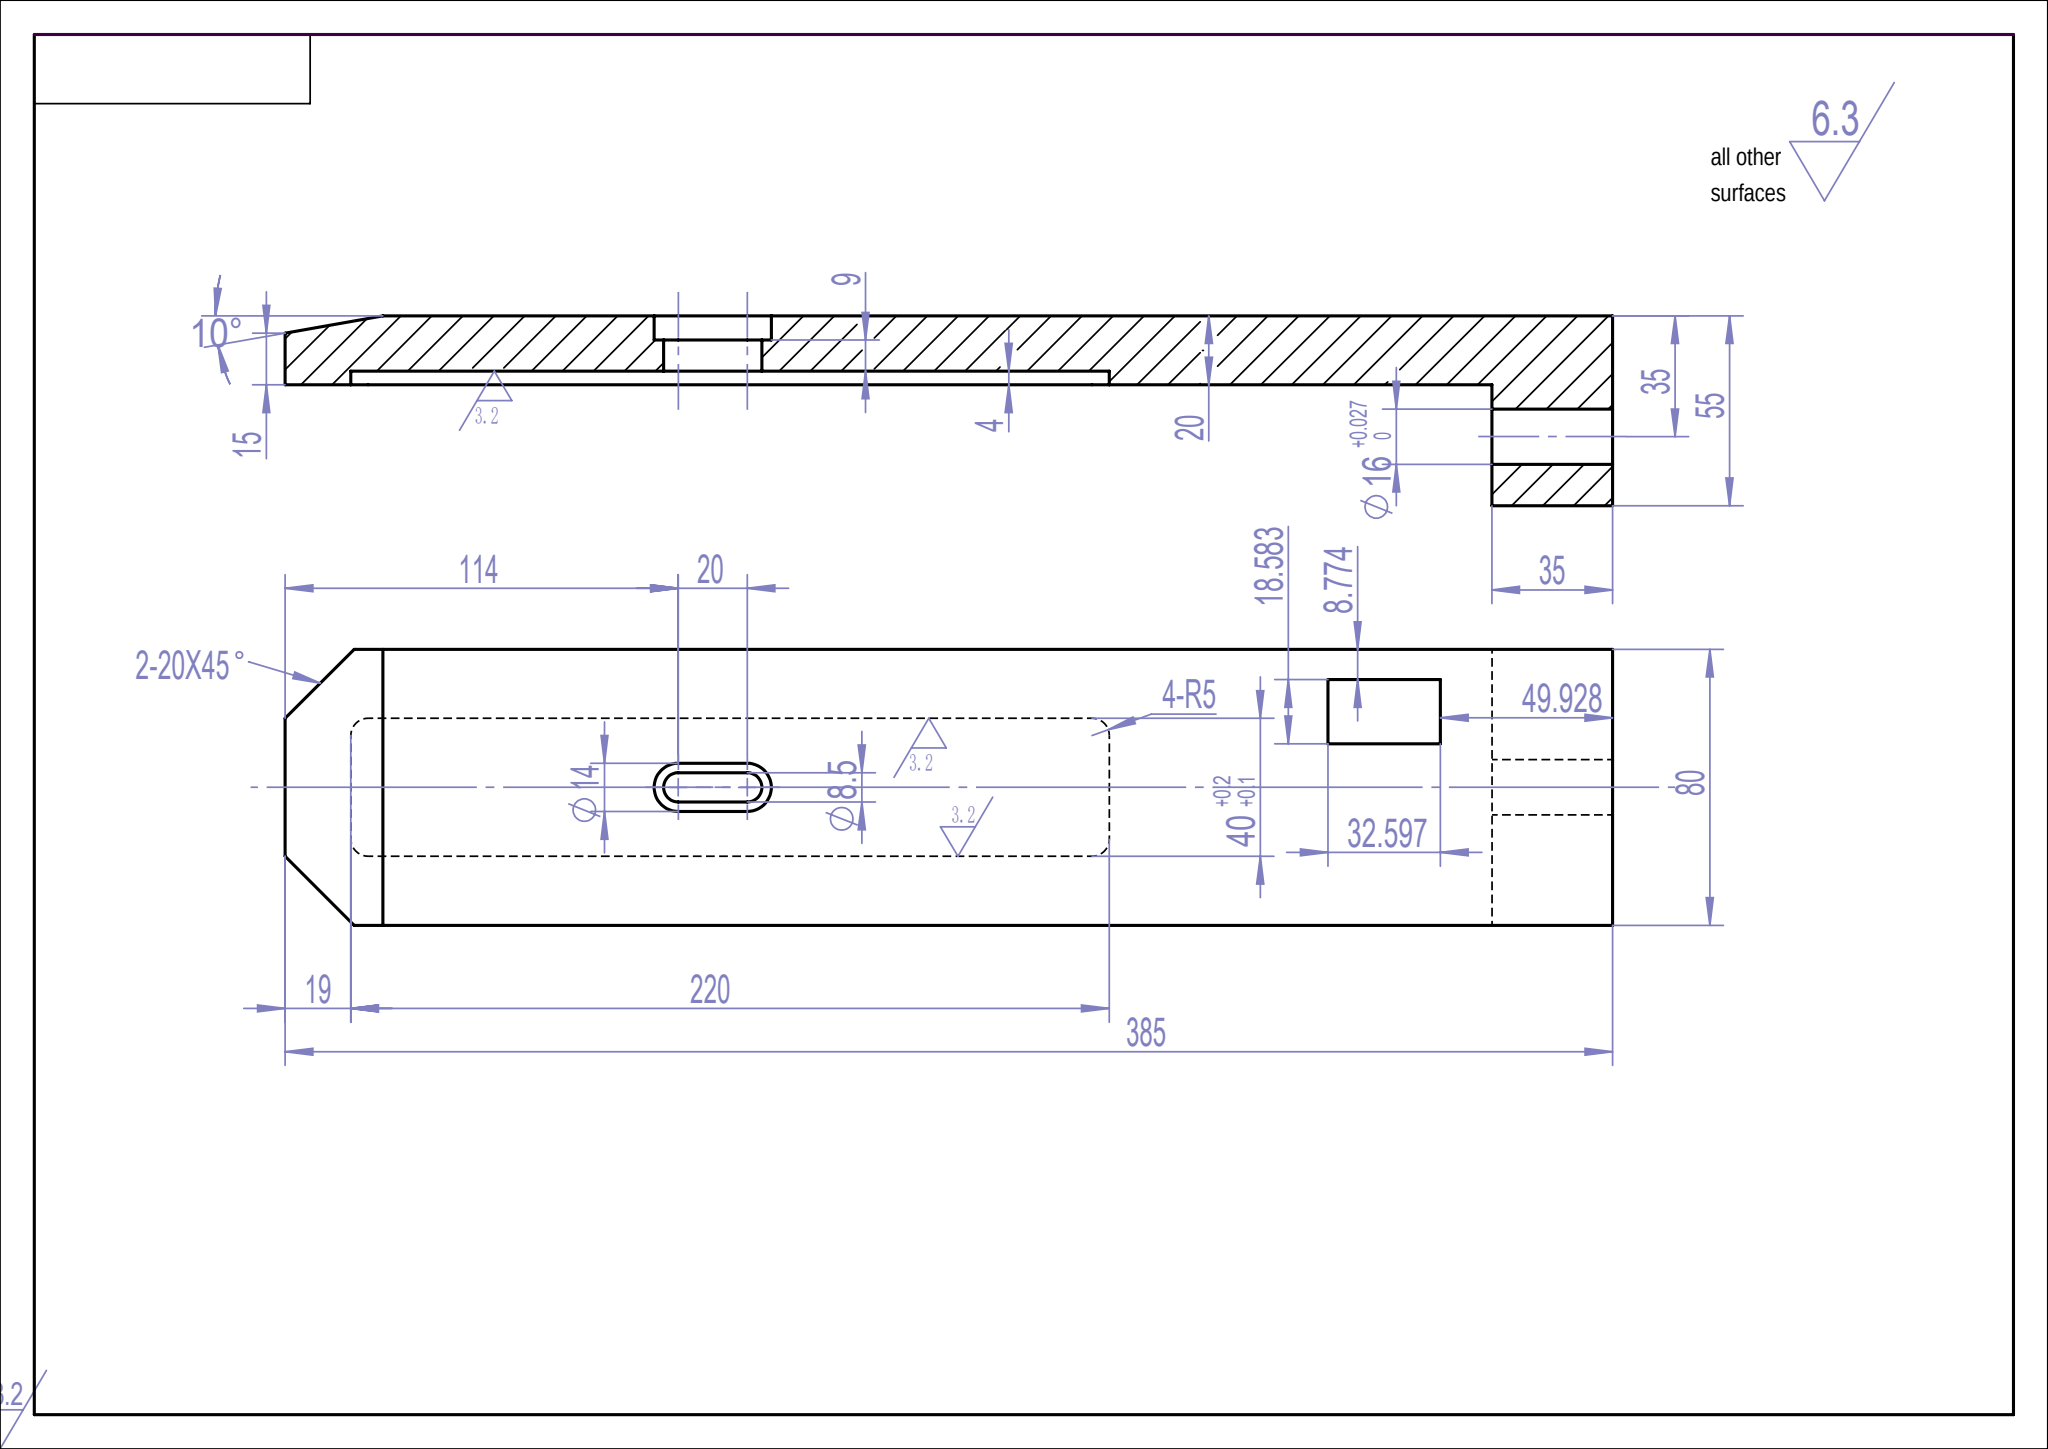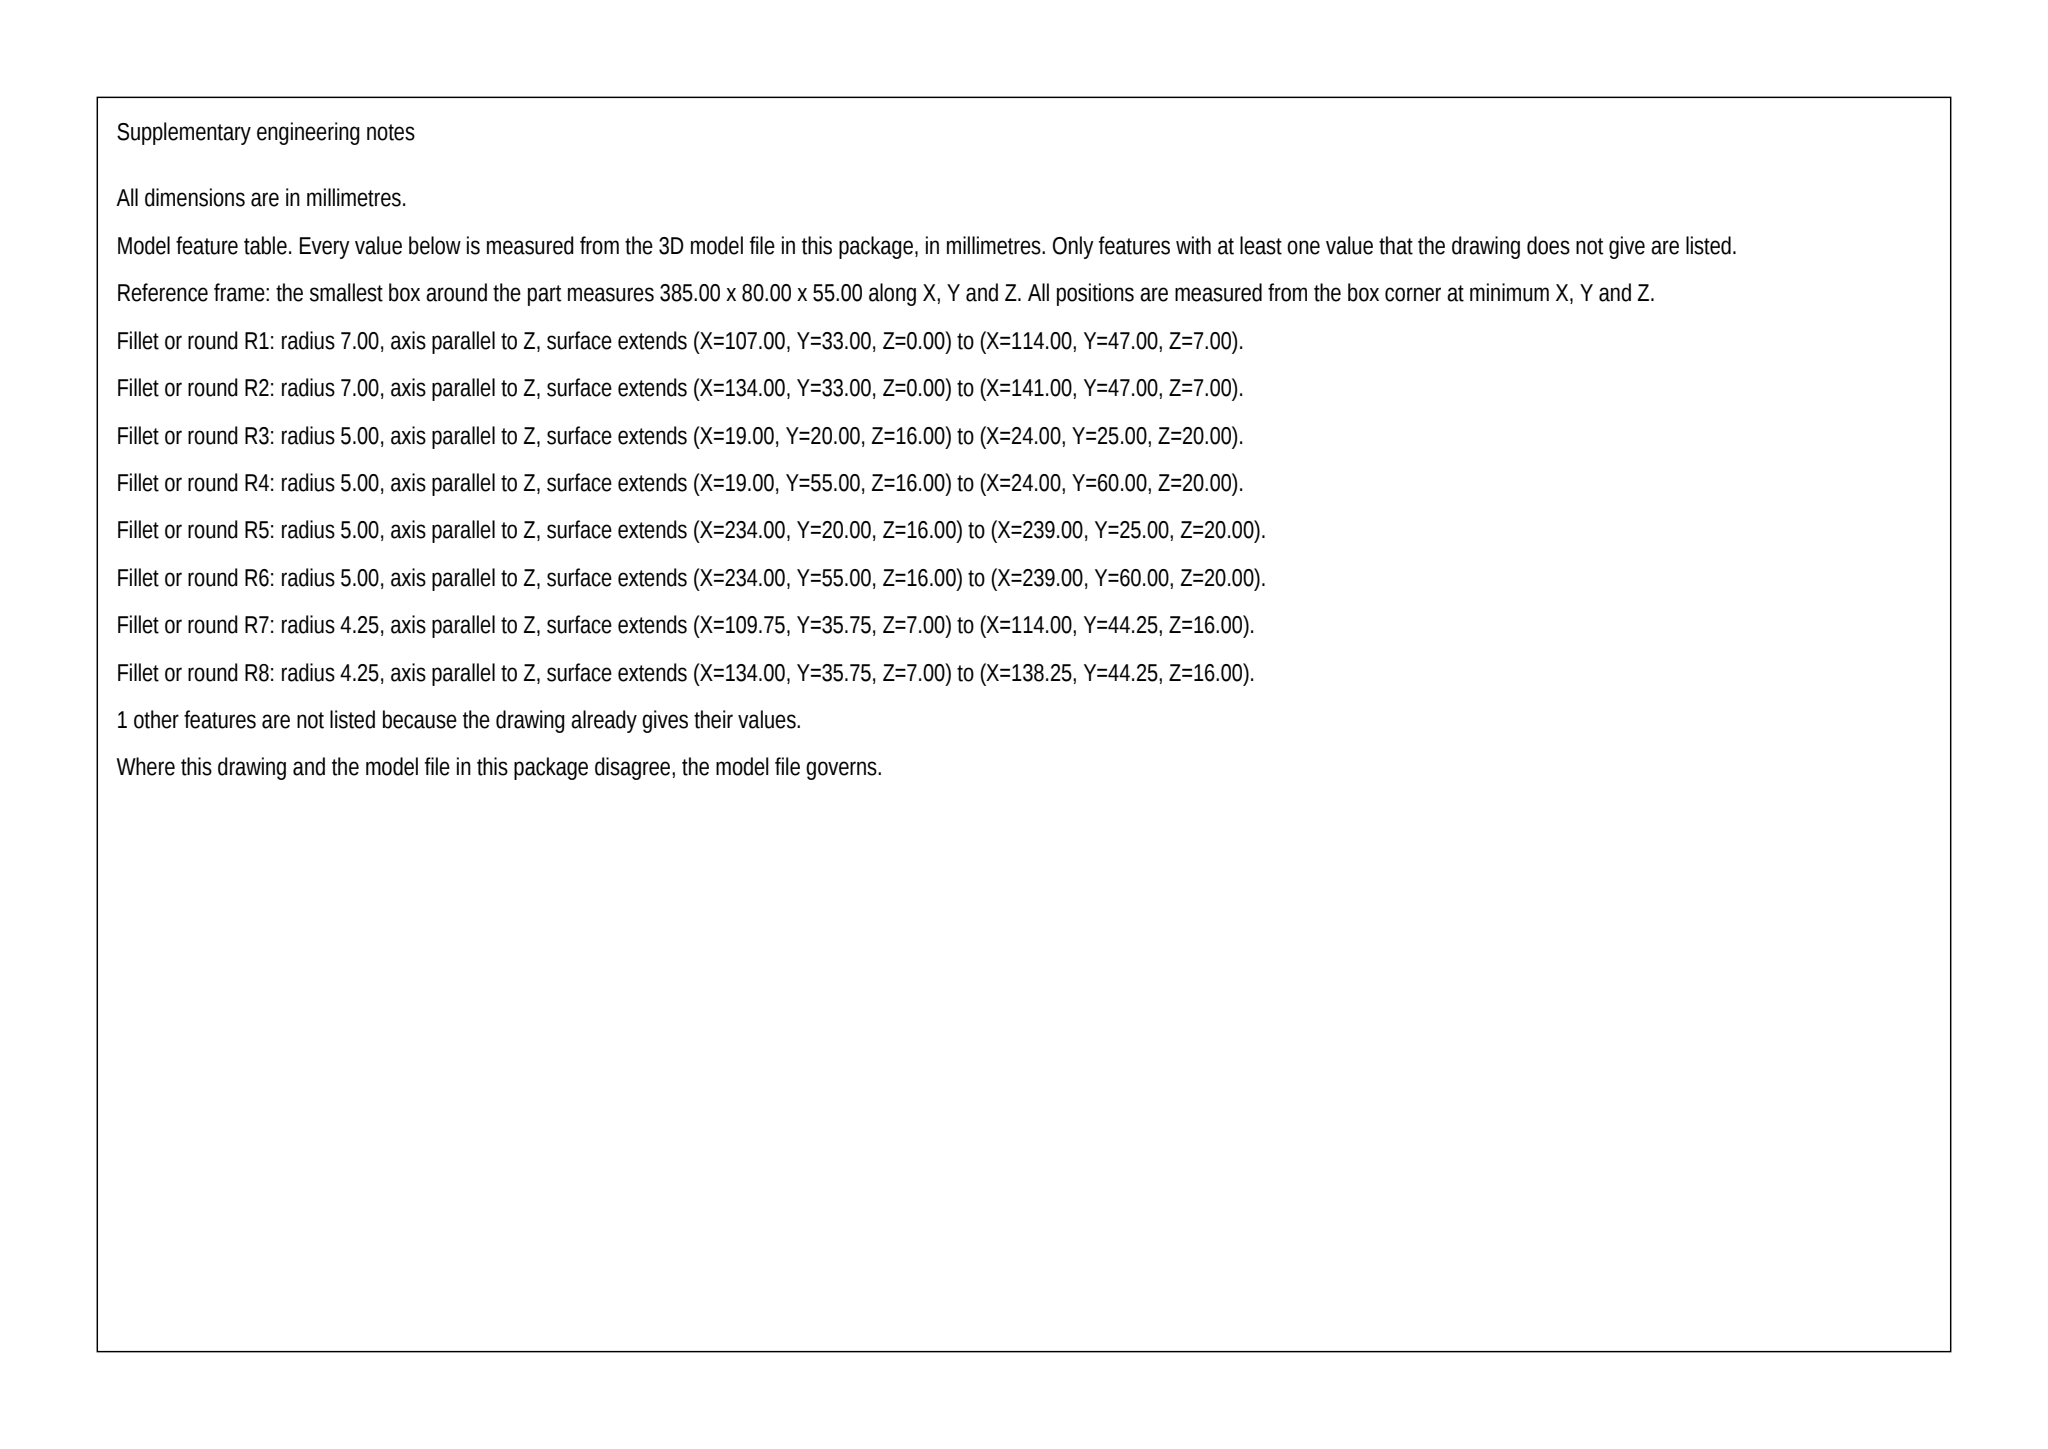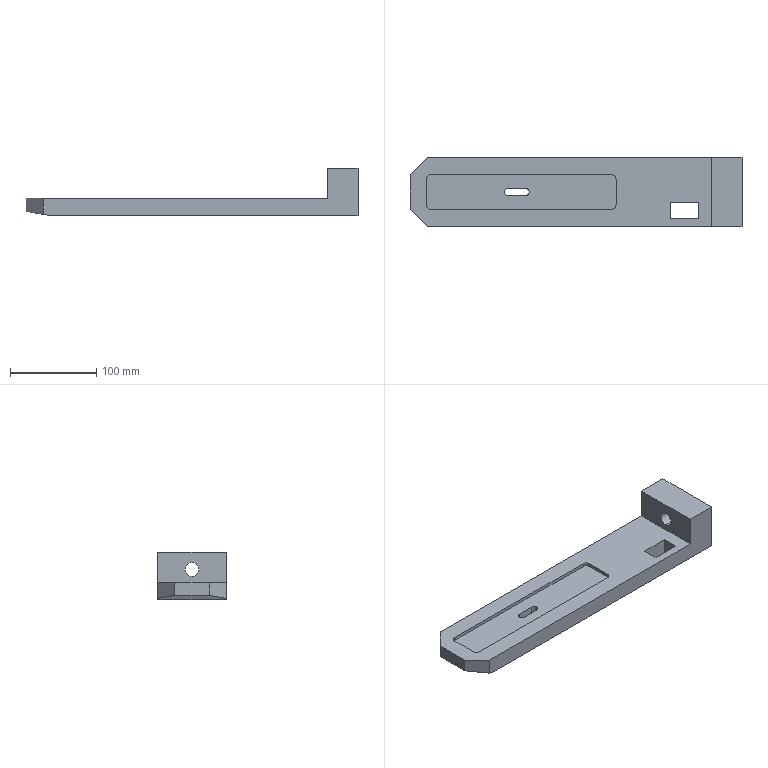Part | SolidWorks | mm | 1 solid | 37 faces | box 385 x 80 x 55 mm | volume 642493 mm3 | plane 25 | cylinder 12 | commonest cylinder face diameters 10 x4 14 x3 8.5 x3 16.024 x2
build123d program:
from build123d import *

# Parameters (mm, degrees)
SKETCH1_W           = 385
SKETCH1_H           = 80
BOSS_EXTRUDE1_DEPTH = 55
SKETCH2_W           = 350
SKETCH2_H           = 80
CUT_EXTRUDE1_DEPTH  = 35
CUT_EXTRUDE2_DEPTH  = 85
SKETCH4_R           = 8.012
CUT_EXTRUDE3_DEPTH  = 85
CHAMFER2_SIZE       = 20
CUT_EXTRUDE4_DEPTH  = 4
CUT_EXTRUDE5_DEPTH  = 9
CUT_EXTRUDE6_DEPTH  = 9
SKETCH8_W           = 32.597
SKETCH8_H           = 18.583
CUT_EXTRUDE7_DEPTH  = 92


with BuildPart() as part:
    # Sketch1 → Boss-Extrude1 (new body)
    with BuildSketch(Plane.XY):
        with Locations((131.989, -14.263)):
            Rectangle(SKETCH1_W, SKETCH1_H)
    extrude(amount=BOSS_EXTRUDE1_DEPTH)

    # Sketch2 → Cut-Extrude1 (cut)
    with BuildSketch(Plane.XY.offset(55)):
        with Locations((114.489, -14.263)):
            Rectangle(SKETCH2_W, SKETCH2_H)
    extrude(amount=-CUT_EXTRUDE1_DEPTH, mode=Mode.SUBTRACT)

    # Sketch3 → Cut-Extrude2 (cut)
    with BuildSketch(Plane(origin=(0, 25.737, 0), x_dir=(1, 0, 0), z_dir=(0, 1, 0))):
        Polygon((-60.511, -5), (-32.154, 0), (-60.511, 0), align=None)
    extrude(amount=-CUT_EXTRUDE2_DEPTH, mode=Mode.SUBTRACT)

    # Sketch4 → Cut-Extrude3 (cut)
    with BuildSketch(Plane(origin=(324.489, 0, 0), x_dir=(0, 0, -1), z_dir=(1, 0, 0))):
        with Locations((-35, -14.263)):
            Circle(SKETCH4_R)
    extrude(amount=-CUT_EXTRUDE3_DEPTH, mode=Mode.SUBTRACT)

    # Chamfer2
    chamfer2_edges = [part.edges().sort_by_distance(p)[0] for p in [
        (-60.511, 25.737, 12.5),
        (-60.511, -54.263, 12.5),
    ]]
    chamfer(chamfer2_edges, length=CHAMFER2_SIZE)

    # Sketch5 → Cut-Extrude4 (cut)
    with BuildSketch(Plane.XY.offset(20)):
        with BuildLine():
            Line((-36.511, 5.737), (173.489, 5.737))
            ThreePointArc((173.489, 5.737), (177.025, 4.272), (178.489, 0.7367))
            Line((178.489, 0.7367), (178.489, -29.263))
            ThreePointArc((178.489, -29.263), (177.025, -32.799), (173.489, -34.263))
            Line((173.489, -34.263), (-36.511, -34.263))
            ThreePointArc((-36.511, -34.263), (-40.046, -32.799), (-41.511, -29.263))
            Line((-41.511, -29.263), (-41.511, 0.7367))
            ThreePointArc((-41.511, 0.7367), (-40.046, 4.272), (-36.511, 5.737))
        make_face()
    extrude(amount=-CUT_EXTRUDE4_DEPTH, mode=Mode.SUBTRACT)

    # Sketch6 → Cut-Extrude5 (cut)
    with BuildSketch(Plane.XY.offset(16)):
        with BuildLine():
            Line((53.489, -10.013), (73.489, -10.013))
            ThreePointArc((73.489, -10.013), (77.739, -14.263), (73.489, -18.513))
            Line((73.489, -18.513), (53.489, -18.513))
            ThreePointArc((53.489, -18.513), (49.239, -14.263), (53.489, -10.013))
        make_face()
    extrude(amount=-CUT_EXTRUDE5_DEPTH, mode=Mode.SUBTRACT)

    # Sketch7 → Cut-Extrude6 (cut)
    with BuildSketch(Plane.XY.offset(7)):
        with BuildLine():
            Line((53.489, -7.263), (73.489, -7.263))
            ThreePointArc((73.489, -7.263), (80.489, -14.263), (73.489, -21.263))
            Line((73.489, -21.263), (53.489, -21.263))
            ThreePointArc((53.489, -21.263), (46.489, -14.263), (53.489, -7.263))
        make_face()
    extrude(amount=-CUT_EXTRUDE6_DEPTH, mode=Mode.SUBTRACT)

    # Sketch8 → Cut-Extrude7 (cut)
    with BuildSketch(Plane.XY.offset(20)):
        with Locations((258.263, -36.197)):
            Rectangle(SKETCH8_W, SKETCH8_H)
    extrude(amount=-CUT_EXTRUDE7_DEPTH, mode=Mode.SUBTRACT)


solid = part.part